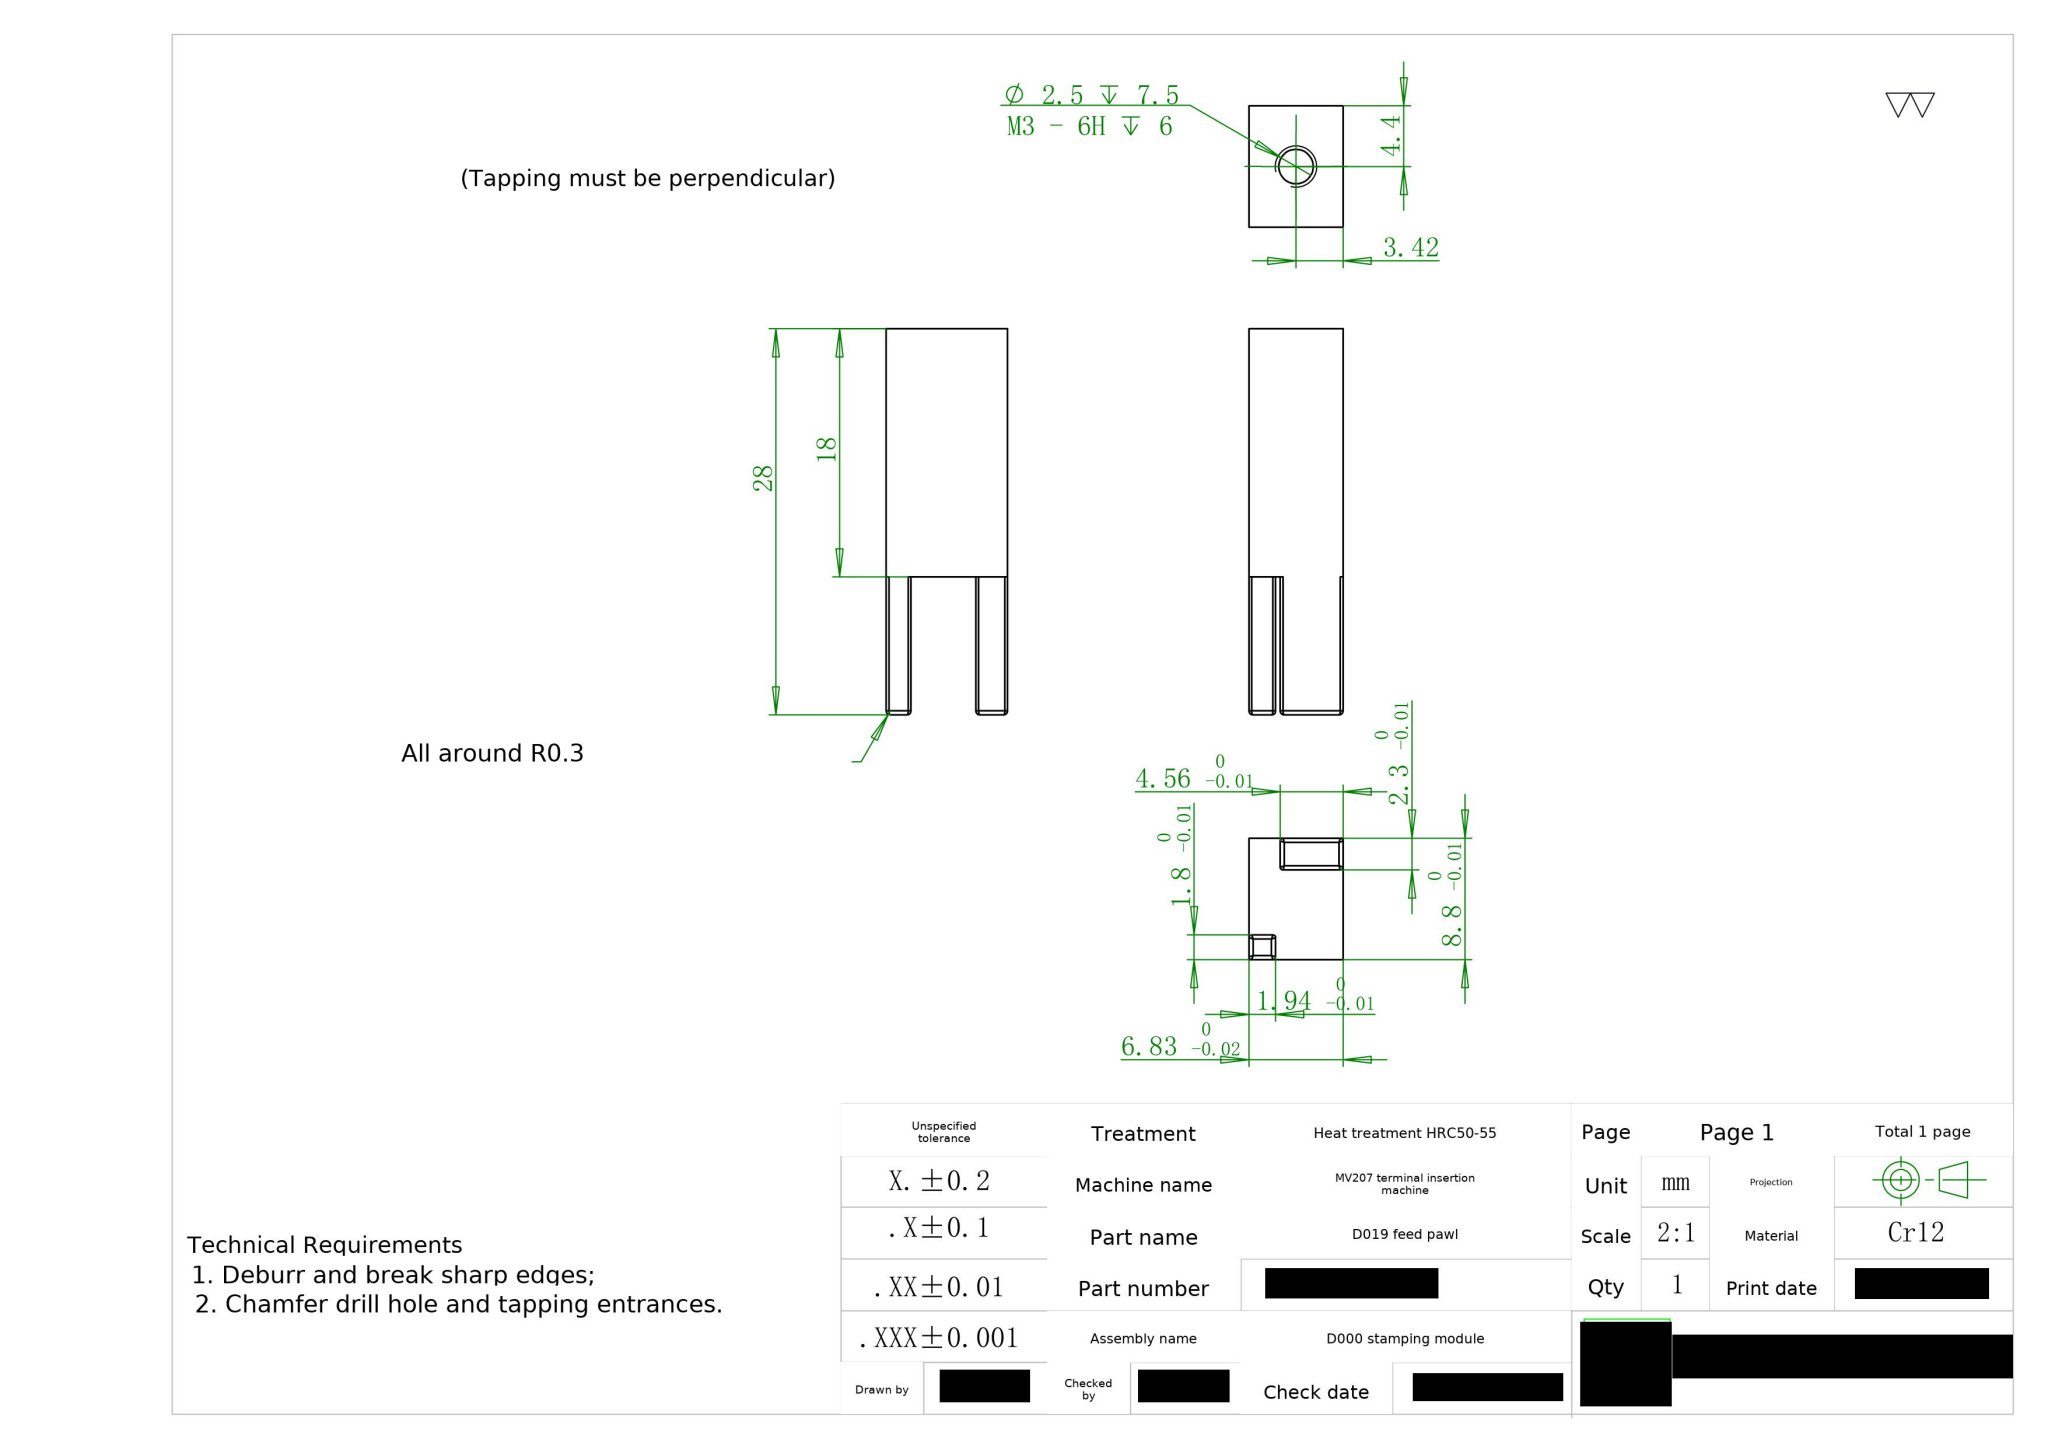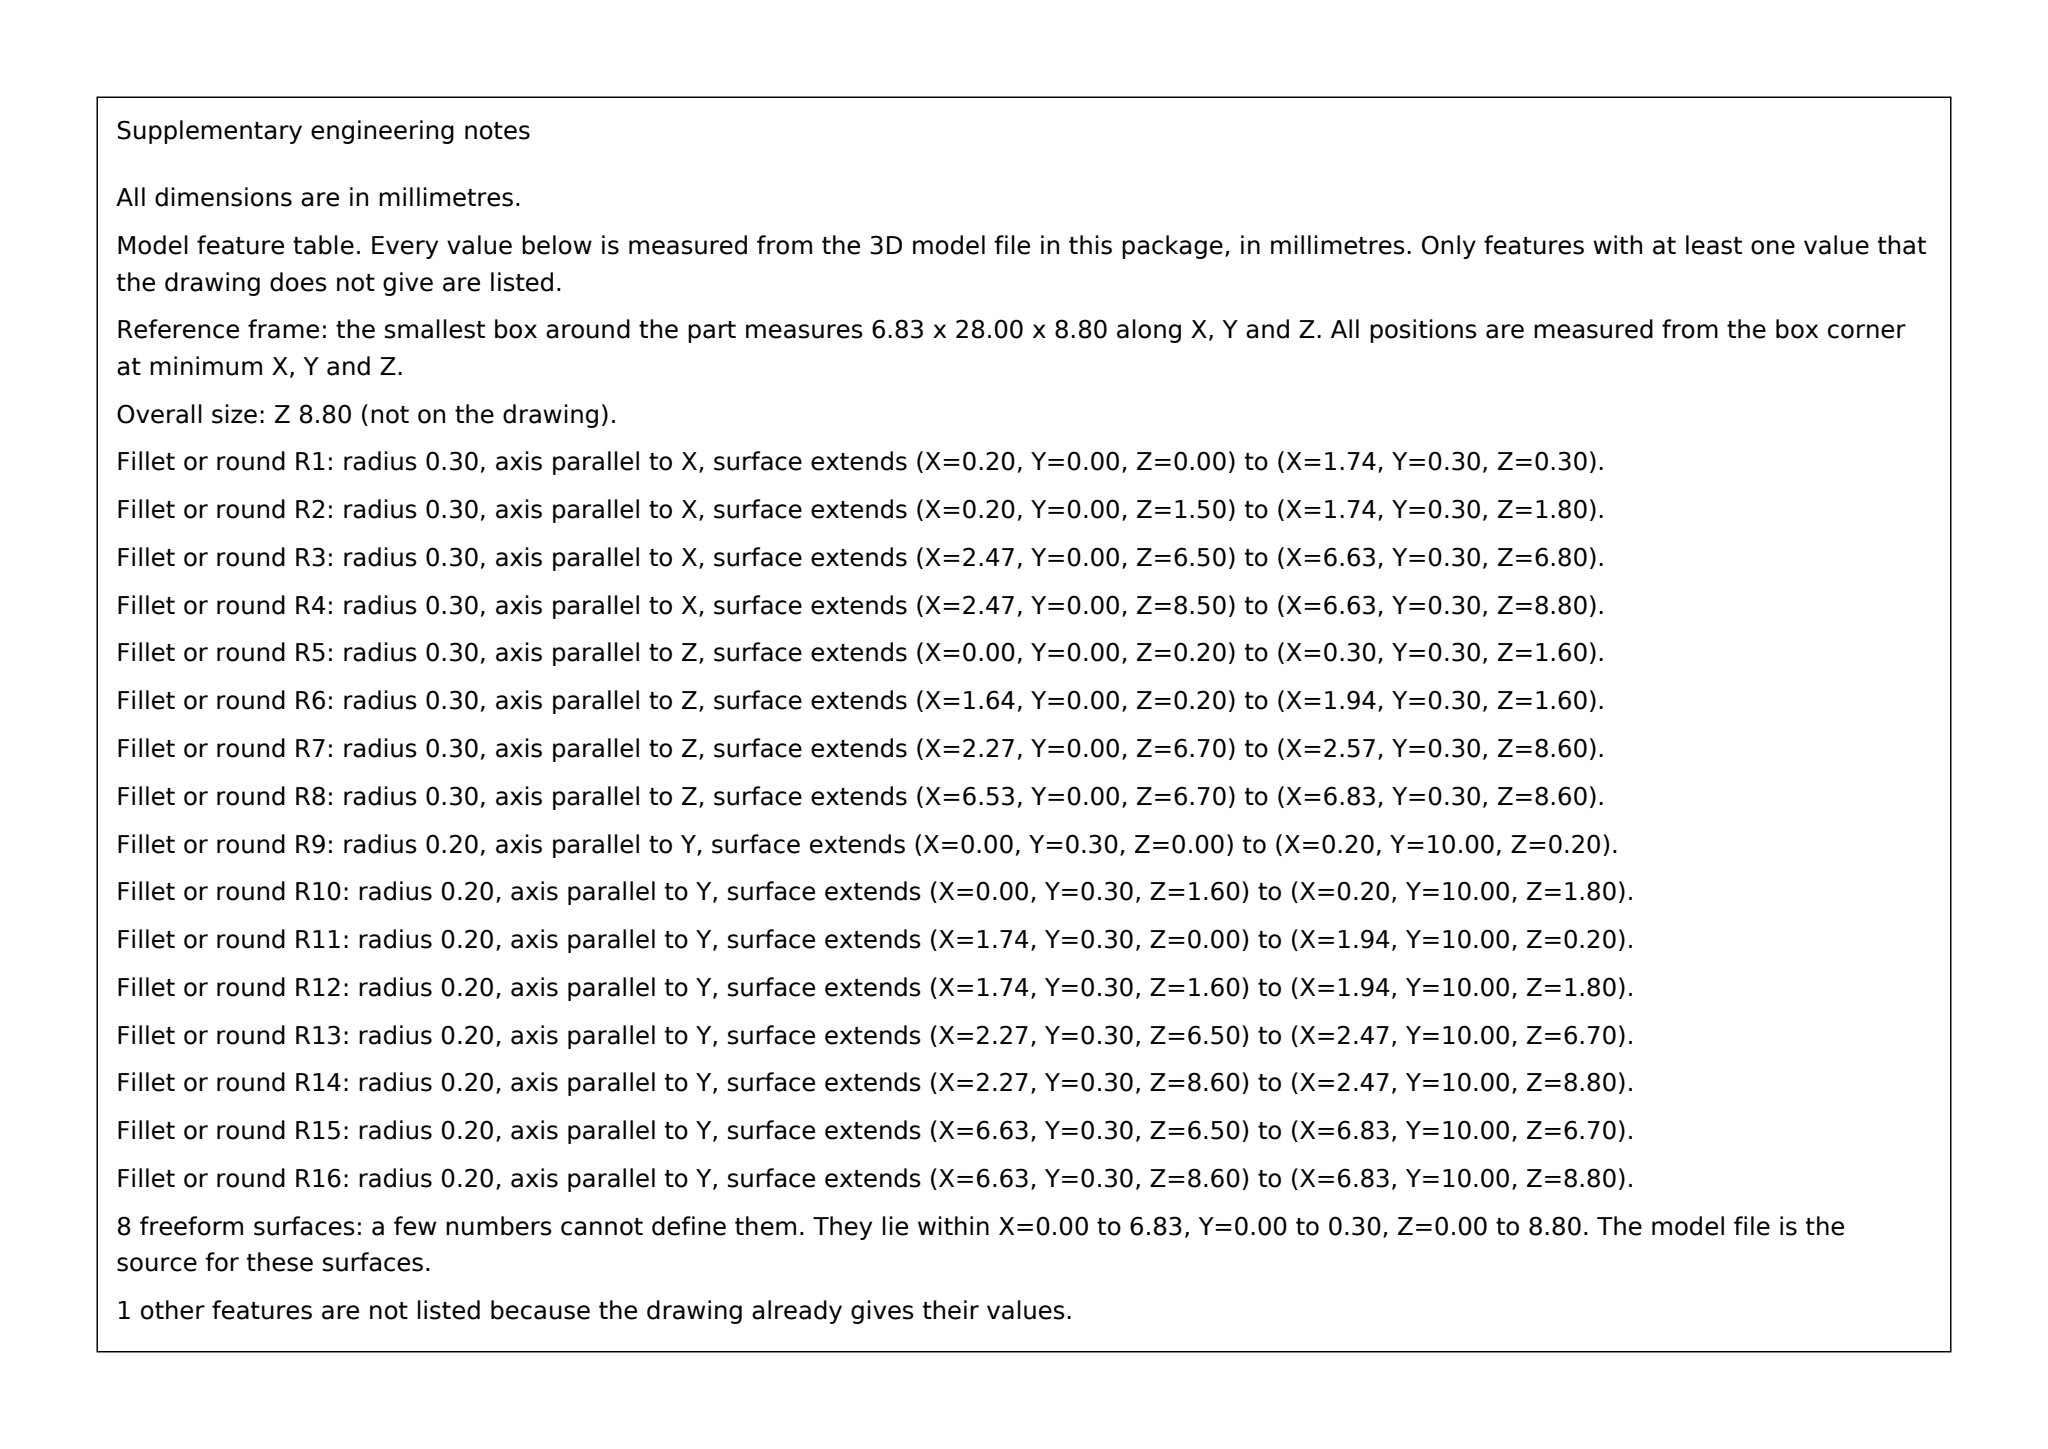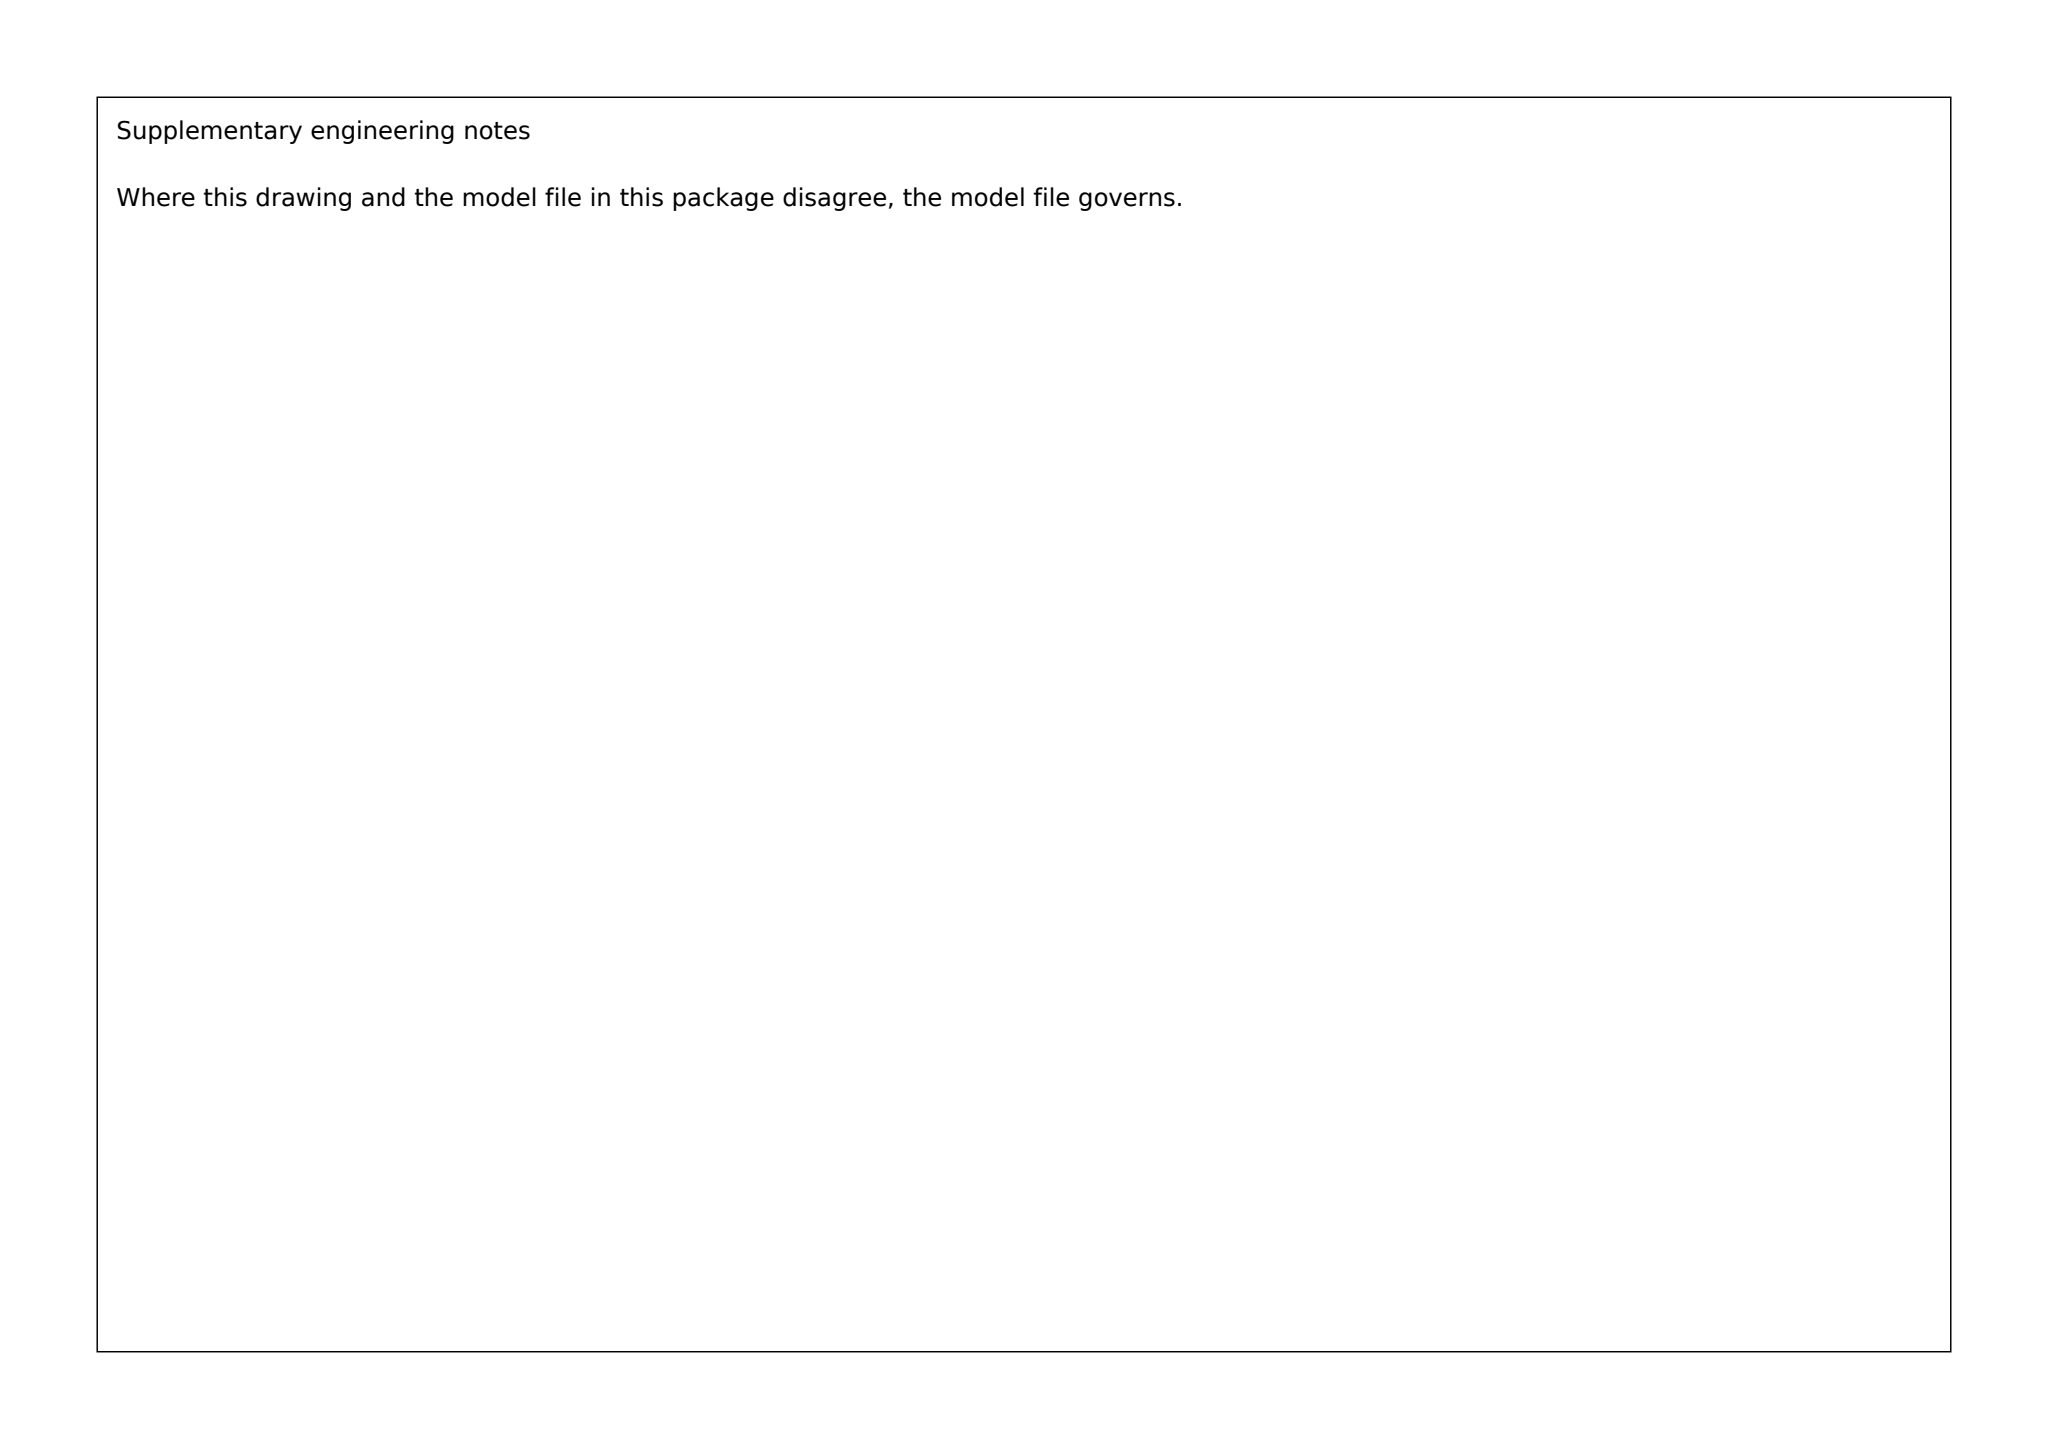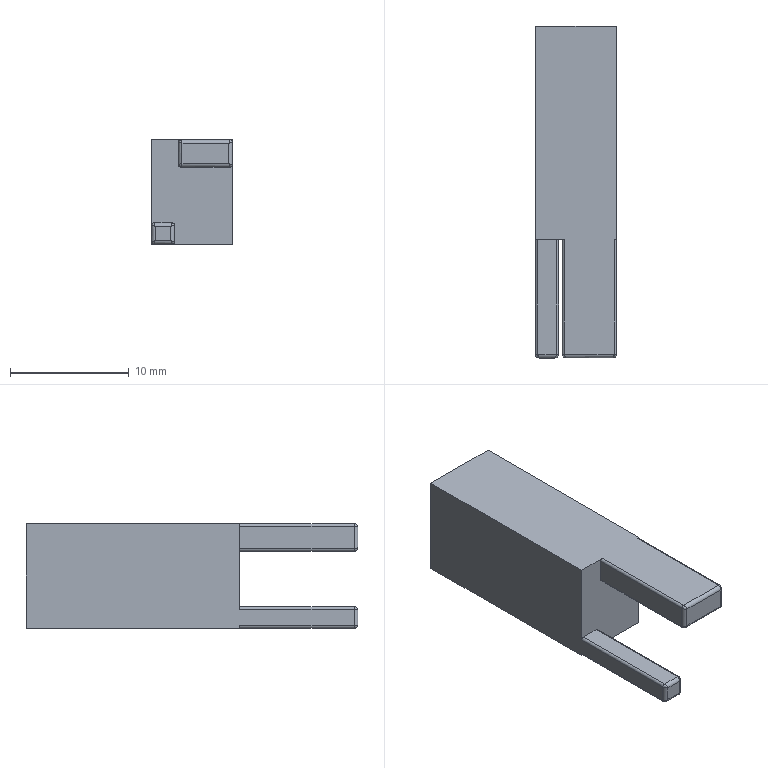Part | SolidWorks | mm | material Cr12 | 1 solid | 42 faces | box 6.83 x 28 x 8.8 mm | volume 1183 mm3 | cylinder 18 | plane 14 | spline 8 | cone 2 | commonest cylinder face diameters 0.6 x8 0.4 x8 2.5 x2